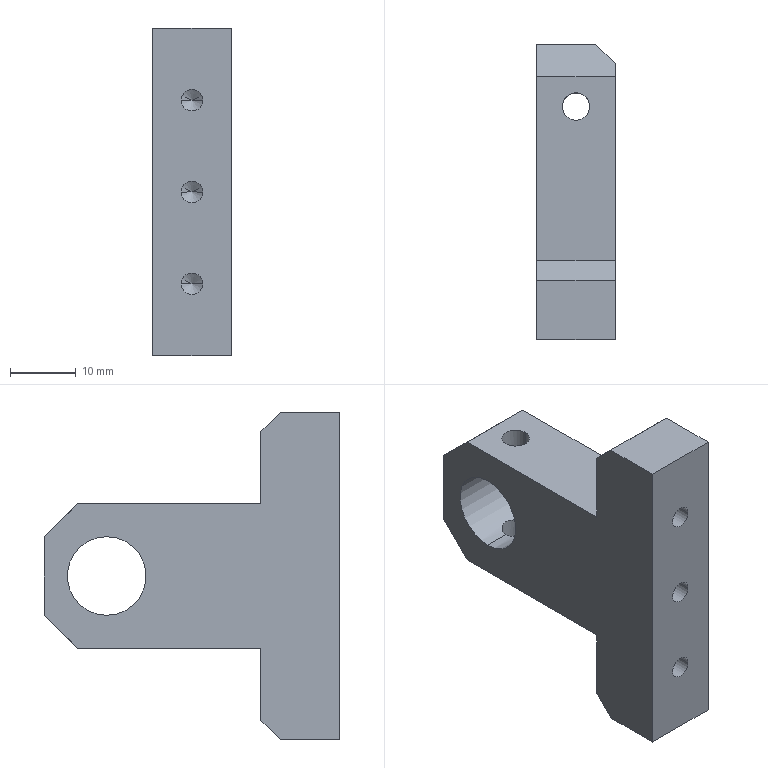Component | SolidWorks | 009BearingHousing-1 | 1 solid | 33 faces | box 12 x 45 x 50 mm | volume 13675 mm3 | plane 15 | cylinder 12 | cone 6 | commonest cylinder face diameters 3.3 x6 4.2 x4 12 x2
build123d program:
from build123d import *

# Parameters (mm, degrees)
SKETCH1_W             = 50
SKETCH1_H             = 45
BOSS_EXTRUDE1_DEPTH   = 12
M4_TAPPED_HOLE1_D     = 3.3
M4_TAPPED_HOLE1_DEPTH = 10.1
M4_TAPPED_HOLE1_TIP   = 0.9914
SKETCH4_R             = 6
CUT_EXTRUDE1_DEPTH    = 36.711
SKETCH5_W             = 14
SKETCH5_H             = 33
CUT_EXTRUDE2_DEPTH    = 36.711
M5_TAPPED_HOLE2_D     = 4.2
CHAMFER1_SIZE         = 5
CHAMFER2_SIZE         = 3
CHAMFER3_SIZE         = 3


with BuildPart() as part:
    # Sketch1 → Boss-Extrude1 (new body)
    with BuildSketch(Plane.XY):
        Rectangle(SKETCH1_W, SKETCH1_H)
    extrude(amount=BOSS_EXTRUDE1_DEPTH)

    # M4 Tapped Hole1
    with Locations(Plane(origin=(0, -22.5, 0), x_dir=(-1, 0, 0), z_dir=(0, -1, 0))):
        with Locations((0, -6), (14, -6), (-14, -6)):
            Hole(M4_TAPPED_HOLE1_D / 2, depth=M4_TAPPED_HOLE1_DEPTH)
            with Locations((0, 0, -(M4_TAPPED_HOLE1_DEPTH + M4_TAPPED_HOLE1_TIP / 2))):  # 118° drill point
                Cone(0, M4_TAPPED_HOLE1_D / 2, M4_TAPPED_HOLE1_TIP, mode=Mode.SUBTRACT)

    # Sketch4 → Cut-Extrude1 (cut, through all)
    with BuildSketch(Plane.XY.offset(12)):
        with Locations((0, 13)):
            Circle(SKETCH4_R)
    extrude(amount=-CUT_EXTRUDE1_DEPTH, mode=Mode.SUBTRACT)

    # Sketch5 → Cut-Extrude2 (cut, through all)
    with BuildSketch(Plane.XY.offset(12)):
        with Locations((-18, 6)):
            Rectangle(SKETCH5_W, SKETCH5_H)
        with Locations((18, 6)):
            Rectangle(SKETCH5_W, SKETCH5_H)
    extrude(amount=-CUT_EXTRUDE2_DEPTH, mode=Mode.SUBTRACT)

    # M5 Tapped Hole2 (through all)
    with Locations(Plane(origin=(11, 0, 0), x_dir=(0, 0, -1), z_dir=(1, 0, 0))):
        with Locations((-6, 13)):
            Hole(M5_TAPPED_HOLE2_D / 2)

    # Chamfer1
    chamfer1_edges = [part.edges().sort_by_distance(p)[0] for p in [
        (-11, 22.5, 6),
        (11, 22.5, 6),
    ]]
    chamfer(chamfer1_edges, length=CHAMFER1_SIZE)

    # Chamfer2
    chamfer2_edges = [part.edges().sort_by_distance(p)[0] for p in [
        (-25, -10.5, 6),
        (25, -10.5, 6),
    ]]
    chamfer(chamfer2_edges, length=CHAMFER2_SIZE)

    # Chamfer3
    chamfer3_edges = [part.edges().sort_by_distance(p)[0] for p in [
        (0, 22.5, 12),
    ]]
    chamfer(chamfer3_edges, length=CHAMFER3_SIZE)


solid = part.part

# Placed as in the assembly
solid = solid.moved(Location((-9.24, 61.679, 11), (0, 90, 0)))